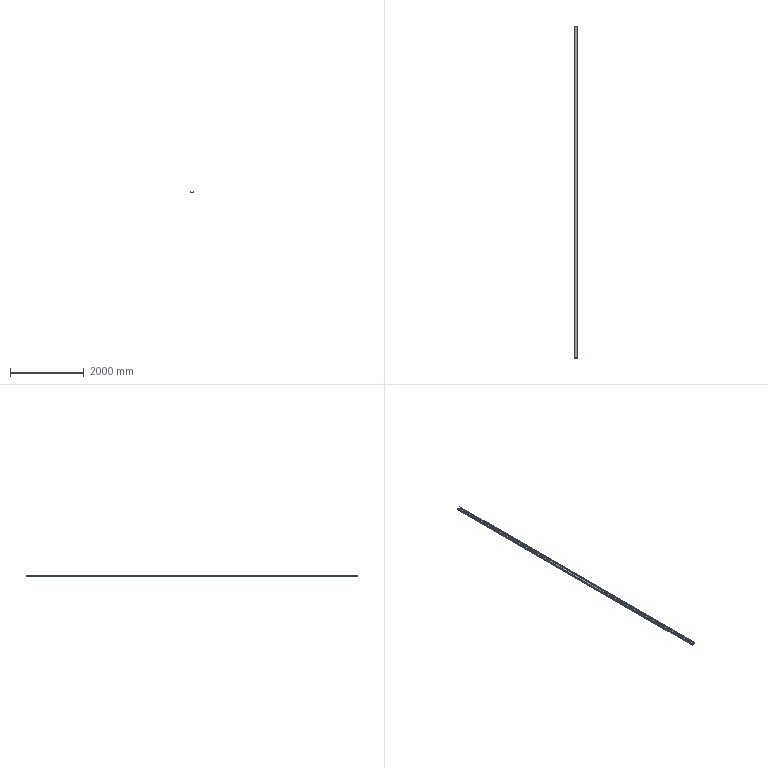Component | NX | CHUNSHUIJINCAO_CAOGANG1 | 1 solid | 10 faces | box 100 x 9000 x 48 mm | volume 11303100 mm3 | plane 10
STEP:
#1=CARTESIAN_POINT('',(0.,0.,0.));
#2=DIRECTION('',(0.,0.,1.));
#3=DIRECTION('',(1.,0.,0.));
#4=AXIS2_PLACEMENT_3D('',#1,#2,#3);
#5=CARTESIAN_POINT('',(2850.,250.,8375.));
#6=VERTEX_POINT('',#5);
#7=CARTESIAN_POINT('',(2850.,250.,8327.));
#8=VERTEX_POINT('',#7);
#9=CARTESIAN_POINT('',(2850.,250.,8327.));
#10=DIRECTION('',(-0.,0.,-1.));
#11=VECTOR('',#10,1.);
#12=LINE('',#9,#11);
#13=CARTESIAN_POINT('',(2850.,150.,8327.));
#14=DIRECTION('',(-1.,0.,0.));
#15=DIRECTION('',(-0.,0.,-1.));
#16=AXIS2_PLACEMENT_3D('',#13,#14,#15);
#17=PLANE('',#16);
#18=CARTESIAN_POINT('',(0.,-100.));
#19=DIRECTION('',(1.,0.));
#20=VECTOR('',#19,1.);
#21=LINE('',#18,#20);
#22=(GEOMETRIC_REPRESENTATION_CONTEXT(2)PARAMETRIC_REPRESENTATION_CONTEXT()REPRESENTATION_CONTEXT('',''));
#23=DEFINITIONAL_REPRESENTATION('',(#21),#22);
#24=PCURVE('',#17,#23);
#25=CARTESIAN_POINT('',(2900.,250.,8351.));
#26=DIRECTION('',(0.,1.,0.));
#27=DIRECTION('',(-1.,0.,0.));
#28=AXIS2_PLACEMENT_3D('',#25,#26,#27);
#29=PLANE('',#28);
#30=CARTESIAN_POINT('',(50.,-24.));
#31=DIRECTION('',(0.,-1.));
#32=VECTOR('',#31,1.);
#33=LINE('',#30,#32);
#34=(GEOMETRIC_REPRESENTATION_CONTEXT(2)PARAMETRIC_REPRESENTATION_CONTEXT()REPRESENTATION_CONTEXT('',''));
#35=DEFINITIONAL_REPRESENTATION('',(#33),#34);
#36=PCURVE('',#29,#35);
#37=SURFACE_CURVE('',#12,(#24,#36),.PCURVE_S1.);
#38=EDGE_CURVE('',#6,#8,#37,.T.);
#39=ORIENTED_EDGE('',*,*,#38,.F.);
#40=CARTESIAN_POINT('',(2850.,9250.,8375.));
#41=VERTEX_POINT('',#40);
#42=CARTESIAN_POINT('',(2850.,150.,8375.));
#43=DIRECTION('',(0.,1.,0.));
#44=VECTOR('',#43,1.);
#45=LINE('',#42,#44);
#46=CARTESIAN_POINT('',(-48.,0.));
#47=DIRECTION('',(0.,-1.));
#48=VECTOR('',#47,1.);
#49=LINE('',#46,#48);
#50=(GEOMETRIC_REPRESENTATION_CONTEXT(2)PARAMETRIC_REPRESENTATION_CONTEXT()REPRESENTATION_CONTEXT('',''));
#51=DEFINITIONAL_REPRESENTATION('',(#49),#50);
#52=PCURVE('',#17,#51);
#53=CARTESIAN_POINT('',(2850.,150.,8375.));
#54=DIRECTION('',(0.,0.,1.));
#55=DIRECTION('',(0.,-1.,0.));
#56=AXIS2_PLACEMENT_3D('',#53,#54,#55);
#57=PLANE('',#56);
#58=CARTESIAN_POINT('',(0.,0.));
#59=DIRECTION('',(-1.,0.));
#60=VECTOR('',#59,1.);
#61=LINE('',#58,#60);
#62=(GEOMETRIC_REPRESENTATION_CONTEXT(2)PARAMETRIC_REPRESENTATION_CONTEXT()REPRESENTATION_CONTEXT('',''));
#63=DEFINITIONAL_REPRESENTATION('',(#61),#62);
#64=PCURVE('',#57,#63);
#65=SURFACE_CURVE('',#45,(#52,#64),.PCURVE_S1.);
#66=EDGE_CURVE('',#6,#41,#65,.T.);
#67=ORIENTED_EDGE('',*,*,#66,.T.);
#68=CARTESIAN_POINT('',(2850.,9250.,8327.));
#69=VERTEX_POINT('',#68);
#70=CARTESIAN_POINT('',(2850.,9250.,8327.));
#71=DIRECTION('',(0.,0.,1.));
#72=VECTOR('',#71,1.);
#73=LINE('',#70,#72);
#74=CARTESIAN_POINT('',(0.,-9100.));
#75=DIRECTION('',(-1.,0.));
#76=VECTOR('',#75,1.);
#77=LINE('',#74,#76);
#78=(GEOMETRIC_REPRESENTATION_CONTEXT(2)PARAMETRIC_REPRESENTATION_CONTEXT()REPRESENTATION_CONTEXT('',''));
#79=DEFINITIONAL_REPRESENTATION('',(#77),#78);
#80=PCURVE('',#17,#79);
#81=CARTESIAN_POINT('',(2900.,9250.,8351.));
#82=DIRECTION('',(0.,-1.,0.));
#83=DIRECTION('',(1.,0.,0.));
#84=AXIS2_PLACEMENT_3D('',#81,#82,#83);
#85=PLANE('',#84);
#86=CARTESIAN_POINT('',(-50.,-24.));
#87=DIRECTION('',(0.,1.));
#88=VECTOR('',#87,1.);
#89=LINE('',#86,#88);
#90=(GEOMETRIC_REPRESENTATION_CONTEXT(2)PARAMETRIC_REPRESENTATION_CONTEXT()REPRESENTATION_CONTEXT('',''));
#91=DEFINITIONAL_REPRESENTATION('',(#89),#90);
#92=PCURVE('',#85,#91);
#93=SURFACE_CURVE('',#73,(#80,#92),.PCURVE_S1.);
#94=EDGE_CURVE('',#69,#41,#93,.T.);
#95=ORIENTED_EDGE('',*,*,#94,.F.);
#96=CARTESIAN_POINT('',(2850.,150.,8327.));
#97=DIRECTION('',(0.,1.,0.));
#98=VECTOR('',#97,1.);
#99=LINE('',#96,#98);
#100=CARTESIAN_POINT('',(0.,0.));
#101=DIRECTION('',(0.,-1.));
#102=VECTOR('',#101,1.);
#103=LINE('',#100,#102);
#104=(GEOMETRIC_REPRESENTATION_CONTEXT(2)PARAMETRIC_REPRESENTATION_CONTEXT()REPRESENTATION_CONTEXT('',''));
#105=DEFINITIONAL_REPRESENTATION('',(#103),#104);
#106=PCURVE('',#17,#105);
#107=CARTESIAN_POINT('',(2950.,150.,8327.));
#108=DIRECTION('',(0.,0.,-1.));
#109=DIRECTION('',(0.,1.,0.));
#110=AXIS2_PLACEMENT_3D('',#107,#108,#109);
#111=PLANE('',#110);
#112=CARTESIAN_POINT('',(0.,-100.));
#113=DIRECTION('',(1.,0.));
#114=VECTOR('',#113,1.);
#115=LINE('',#112,#114);
#116=(GEOMETRIC_REPRESENTATION_CONTEXT(2)PARAMETRIC_REPRESENTATION_CONTEXT()REPRESENTATION_CONTEXT('',''));
#117=DEFINITIONAL_REPRESENTATION('',(#115),#116);
#118=PCURVE('',#111,#117);
#119=SURFACE_CURVE('',#99,(#106,#118),.PCURVE_S1.);
#120=EDGE_CURVE('',#8,#69,#119,.T.);
#121=ORIENTED_EDGE('',*,*,#120,.F.);
#122=EDGE_LOOP('',(#39,#67,#95,#121));
#123=FACE_BOUND('',#122,.T.);
#124=ADVANCED_FACE('',(#123),#17,.T.);
#125=CARTESIAN_POINT('',(2858.5,250.,8375.));
#126=VERTEX_POINT('',#125);
#127=CARTESIAN_POINT('',(2850.,250.,8375.));
#128=DIRECTION('',(-1.,0.,0.));
#129=VECTOR('',#128,1.);
#130=LINE('',#127,#129);
#131=CARTESIAN_POINT('',(-100.,0.));
#132=DIRECTION('',(0.,-1.));
#133=VECTOR('',#132,1.);
#134=LINE('',#131,#133);
#135=(GEOMETRIC_REPRESENTATION_CONTEXT(2)PARAMETRIC_REPRESENTATION_CONTEXT()REPRESENTATION_CONTEXT('',''));
#136=DEFINITIONAL_REPRESENTATION('',(#134),#135);
#137=PCURVE('',#57,#136);
#138=CARTESIAN_POINT('',(50.,24.));
#139=DIRECTION('',(1.,0.));
#140=VECTOR('',#139,1.);
#141=LINE('',#138,#140);
#142=(GEOMETRIC_REPRESENTATION_CONTEXT(2)PARAMETRIC_REPRESENTATION_CONTEXT()REPRESENTATION_CONTEXT('',''));
#143=DEFINITIONAL_REPRESENTATION('',(#141),#142);
#144=PCURVE('',#29,#143);
#145=SURFACE_CURVE('',#130,(#137,#144),.PCURVE_S1.);
#146=EDGE_CURVE('',#126,#6,#145,.T.);
#147=ORIENTED_EDGE('',*,*,#146,.F.);
#148=CARTESIAN_POINT('',(2858.5,9250.,8375.));
#149=VERTEX_POINT('',#148);
#150=CARTESIAN_POINT('',(2858.5,150.,8375.));
#151=DIRECTION('',(0.,1.,0.));
#152=VECTOR('',#151,1.);
#153=LINE('',#150,#152);
#154=CARTESIAN_POINT('',(0.,8.5));
#155=DIRECTION('',(-1.,0.));
#156=VECTOR('',#155,1.);
#157=LINE('',#154,#156);
#158=(GEOMETRIC_REPRESENTATION_CONTEXT(2)PARAMETRIC_REPRESENTATION_CONTEXT()REPRESENTATION_CONTEXT('',''));
#159=DEFINITIONAL_REPRESENTATION('',(#157),#158);
#160=PCURVE('',#57,#159);
#161=CARTESIAN_POINT('',(2858.5,150.,8375.));
#162=DIRECTION('',(1.,0.,-0.));
#163=DIRECTION('',(0.,0.,1.));
#164=AXIS2_PLACEMENT_3D('',#161,#162,#163);
#165=PLANE('',#164);
#166=CARTESIAN_POINT('',(0.,0.));
#167=DIRECTION('',(0.,-1.));
#168=VECTOR('',#167,1.);
#169=LINE('',#166,#168);
#170=(GEOMETRIC_REPRESENTATION_CONTEXT(2)PARAMETRIC_REPRESENTATION_CONTEXT()REPRESENTATION_CONTEXT('',''));
#171=DEFINITIONAL_REPRESENTATION('',(#169),#170);
#172=PCURVE('',#165,#171);
#173=SURFACE_CURVE('',#153,(#160,#172),.PCURVE_S1.);
#174=EDGE_CURVE('',#126,#149,#173,.T.);
#175=ORIENTED_EDGE('',*,*,#174,.T.);
#176=CARTESIAN_POINT('',(2850.,9250.,8375.));
#177=DIRECTION('',(1.,0.,0.));
#178=VECTOR('',#177,1.);
#179=LINE('',#176,#178);
#180=CARTESIAN_POINT('',(-9100.,0.));
#181=DIRECTION('',(0.,1.));
#182=VECTOR('',#181,1.);
#183=LINE('',#180,#182);
#184=(GEOMETRIC_REPRESENTATION_CONTEXT(2)PARAMETRIC_REPRESENTATION_CONTEXT()REPRESENTATION_CONTEXT('',''));
#185=DEFINITIONAL_REPRESENTATION('',(#183),#184);
#186=PCURVE('',#57,#185);
#187=CARTESIAN_POINT('',(-50.,24.));
#188=DIRECTION('',(1.,0.));
#189=VECTOR('',#188,1.);
#190=LINE('',#187,#189);
#191=(GEOMETRIC_REPRESENTATION_CONTEXT(2)PARAMETRIC_REPRESENTATION_CONTEXT()REPRESENTATION_CONTEXT('',''));
#192=DEFINITIONAL_REPRESENTATION('',(#190),#191);
#193=PCURVE('',#85,#192);
#194=SURFACE_CURVE('',#179,(#186,#193),.PCURVE_S1.);
#195=EDGE_CURVE('',#41,#149,#194,.T.);
#196=ORIENTED_EDGE('',*,*,#195,.F.);
#197=ORIENTED_EDGE('',*,*,#66,.F.);
#198=EDGE_LOOP('',(#147,#175,#196,#197));
#199=FACE_BOUND('',#198,.T.);
#200=ADVANCED_FACE('',(#199),#57,.T.);
#201=CARTESIAN_POINT('',(2858.5,250.,8332.3));
#202=VERTEX_POINT('',#201);
#203=CARTESIAN_POINT('',(2858.5,250.,8375.));
#204=DIRECTION('',(0.,0.,1.));
#205=VECTOR('',#204,1.);
#206=LINE('',#203,#205);
#207=CARTESIAN_POINT('',(0.,-100.));
#208=DIRECTION('',(1.,0.));
#209=VECTOR('',#208,1.);
#210=LINE('',#207,#209);
#211=(GEOMETRIC_REPRESENTATION_CONTEXT(2)PARAMETRIC_REPRESENTATION_CONTEXT()REPRESENTATION_CONTEXT('',''));
#212=DEFINITIONAL_REPRESENTATION('',(#210),#211);
#213=PCURVE('',#165,#212);
#214=CARTESIAN_POINT('',(41.5,24.));
#215=DIRECTION('',(-0.,1.));
#216=VECTOR('',#215,1.);
#217=LINE('',#214,#216);
#218=(GEOMETRIC_REPRESENTATION_CONTEXT(2)PARAMETRIC_REPRESENTATION_CONTEXT()REPRESENTATION_CONTEXT('',''));
#219=DEFINITIONAL_REPRESENTATION('',(#217),#218);
#220=PCURVE('',#29,#219);
#221=SURFACE_CURVE('',#206,(#213,#220),.PCURVE_S1.);
#222=EDGE_CURVE('',#202,#126,#221,.T.);
#223=ORIENTED_EDGE('',*,*,#222,.F.);
#224=CARTESIAN_POINT('',(2858.5,9250.,8332.3));
#225=VERTEX_POINT('',#224);
#226=CARTESIAN_POINT('',(2858.5,150.,8332.3));
#227=DIRECTION('',(0.,1.,0.));
#228=VECTOR('',#227,1.);
#229=LINE('',#226,#228);
#230=CARTESIAN_POINT('',(-42.7,0.));
#231=DIRECTION('',(0.,-1.));
#232=VECTOR('',#231,1.);
#233=LINE('',#230,#232);
#234=(GEOMETRIC_REPRESENTATION_CONTEXT(2)PARAMETRIC_REPRESENTATION_CONTEXT()REPRESENTATION_CONTEXT('',''));
#235=DEFINITIONAL_REPRESENTATION('',(#233),#234);
#236=PCURVE('',#165,#235);
#237=CARTESIAN_POINT('',(2900.,150.,8332.3));
#238=DIRECTION('',(0.,0.,1.));
#239=DIRECTION('',(0.,-1.,0.));
#240=AXIS2_PLACEMENT_3D('',#237,#238,#239);
#241=PLANE('',#240);
#242=CARTESIAN_POINT('',(0.,-41.5));
#243=DIRECTION('',(-1.,0.));
#244=VECTOR('',#243,1.);
#245=LINE('',#242,#244);
#246=(GEOMETRIC_REPRESENTATION_CONTEXT(2)PARAMETRIC_REPRESENTATION_CONTEXT()REPRESENTATION_CONTEXT('',''));
#247=DEFINITIONAL_REPRESENTATION('',(#245),#246);
#248=PCURVE('',#241,#247);
#249=SURFACE_CURVE('',#229,(#236,#248),.PCURVE_S1.);
#250=EDGE_CURVE('',#202,#225,#249,.T.);
#251=ORIENTED_EDGE('',*,*,#250,.T.);
#252=CARTESIAN_POINT('',(2858.5,9250.,8375.));
#253=DIRECTION('',(-0.,0.,-1.));
#254=VECTOR('',#253,1.);
#255=LINE('',#252,#254);
#256=CARTESIAN_POINT('',(0.,-9100.));
#257=DIRECTION('',(-1.,0.));
#258=VECTOR('',#257,1.);
#259=LINE('',#256,#258);
#260=(GEOMETRIC_REPRESENTATION_CONTEXT(2)PARAMETRIC_REPRESENTATION_CONTEXT()REPRESENTATION_CONTEXT('',''));
#261=DEFINITIONAL_REPRESENTATION('',(#259),#260);
#262=PCURVE('',#165,#261);
#263=CARTESIAN_POINT('',(-41.5,24.));
#264=DIRECTION('',(-0.,-1.));
#265=VECTOR('',#264,1.);
#266=LINE('',#263,#265);
#267=(GEOMETRIC_REPRESENTATION_CONTEXT(2)PARAMETRIC_REPRESENTATION_CONTEXT()REPRESENTATION_CONTEXT('',''));
#268=DEFINITIONAL_REPRESENTATION('',(#266),#267);
#269=PCURVE('',#85,#268);
#270=SURFACE_CURVE('',#255,(#262,#269),.PCURVE_S1.);
#271=EDGE_CURVE('',#149,#225,#270,.T.);
#272=ORIENTED_EDGE('',*,*,#271,.F.);
#273=ORIENTED_EDGE('',*,*,#174,.F.);
#274=EDGE_LOOP('',(#223,#251,#272,#273));
#275=FACE_BOUND('',#274,.T.);
#276=ADVANCED_FACE('',(#275),#165,.T.);
#277=CARTESIAN_POINT('',(2941.5,250.,8332.3));
#278=VERTEX_POINT('',#277);
#279=CARTESIAN_POINT('',(2900.,250.,8332.3));
#280=DIRECTION('',(-1.,0.,0.));
#281=VECTOR('',#280,1.);
#282=LINE('',#279,#281);
#283=CARTESIAN_POINT('',(-100.,0.));
#284=DIRECTION('',(0.,-1.));
#285=VECTOR('',#284,1.);
#286=LINE('',#283,#285);
#287=(GEOMETRIC_REPRESENTATION_CONTEXT(2)PARAMETRIC_REPRESENTATION_CONTEXT()REPRESENTATION_CONTEXT('',''));
#288=DEFINITIONAL_REPRESENTATION('',(#286),#287);
#289=PCURVE('',#241,#288);
#290=CARTESIAN_POINT('',(0.,-18.7));
#291=DIRECTION('',(1.,0.));
#292=VECTOR('',#291,1.);
#293=LINE('',#290,#292);
#294=(GEOMETRIC_REPRESENTATION_CONTEXT(2)PARAMETRIC_REPRESENTATION_CONTEXT()REPRESENTATION_CONTEXT('',''));
#295=DEFINITIONAL_REPRESENTATION('',(#293),#294);
#296=PCURVE('',#29,#295);
#297=SURFACE_CURVE('',#282,(#289,#296),.PCURVE_S1.);
#298=EDGE_CURVE('',#278,#202,#297,.T.);
#299=ORIENTED_EDGE('',*,*,#298,.F.);
#300=CARTESIAN_POINT('',(2941.5,9250.,8332.3));
#301=VERTEX_POINT('',#300);
#302=CARTESIAN_POINT('',(2941.5,150.,8332.3));
#303=DIRECTION('',(0.,1.,0.));
#304=VECTOR('',#303,1.);
#305=LINE('',#302,#304);
#306=CARTESIAN_POINT('',(0.,41.5));
#307=DIRECTION('',(-1.,0.));
#308=VECTOR('',#307,1.);
#309=LINE('',#306,#308);
#310=(GEOMETRIC_REPRESENTATION_CONTEXT(2)PARAMETRIC_REPRESENTATION_CONTEXT()REPRESENTATION_CONTEXT('',''));
#311=DEFINITIONAL_REPRESENTATION('',(#309),#310);
#312=PCURVE('',#241,#311);
#313=CARTESIAN_POINT('',(2941.5,150.,8332.3));
#314=DIRECTION('',(-1.,0.,0.));
#315=DIRECTION('',(-0.,0.,-1.));
#316=AXIS2_PLACEMENT_3D('',#313,#314,#315);
#317=PLANE('',#316);
#318=CARTESIAN_POINT('',(0.,0.));
#319=DIRECTION('',(0.,-1.));
#320=VECTOR('',#319,1.);
#321=LINE('',#318,#320);
#322=(GEOMETRIC_REPRESENTATION_CONTEXT(2)PARAMETRIC_REPRESENTATION_CONTEXT()REPRESENTATION_CONTEXT('',''));
#323=DEFINITIONAL_REPRESENTATION('',(#321),#322);
#324=PCURVE('',#317,#323);
#325=SURFACE_CURVE('',#305,(#312,#324),.PCURVE_S1.);
#326=EDGE_CURVE('',#278,#301,#325,.T.);
#327=ORIENTED_EDGE('',*,*,#326,.T.);
#328=CARTESIAN_POINT('',(2900.,9250.,8332.3));
#329=DIRECTION('',(1.,0.,0.));
#330=VECTOR('',#329,1.);
#331=LINE('',#328,#330);
#332=CARTESIAN_POINT('',(-9100.,0.));
#333=DIRECTION('',(0.,1.));
#334=VECTOR('',#333,1.);
#335=LINE('',#332,#334);
#336=(GEOMETRIC_REPRESENTATION_CONTEXT(2)PARAMETRIC_REPRESENTATION_CONTEXT()REPRESENTATION_CONTEXT('',''));
#337=DEFINITIONAL_REPRESENTATION('',(#335),#336);
#338=PCURVE('',#241,#337);
#339=CARTESIAN_POINT('',(0.,-18.7));
#340=DIRECTION('',(1.,0.));
#341=VECTOR('',#340,1.);
#342=LINE('',#339,#341);
#343=(GEOMETRIC_REPRESENTATION_CONTEXT(2)PARAMETRIC_REPRESENTATION_CONTEXT()REPRESENTATION_CONTEXT('',''));
#344=DEFINITIONAL_REPRESENTATION('',(#342),#343);
#345=PCURVE('',#85,#344);
#346=SURFACE_CURVE('',#331,(#338,#345),.PCURVE_S1.);
#347=EDGE_CURVE('',#225,#301,#346,.T.);
#348=ORIENTED_EDGE('',*,*,#347,.F.);
#349=ORIENTED_EDGE('',*,*,#250,.F.);
#350=EDGE_LOOP('',(#299,#327,#348,#349));
#351=FACE_BOUND('',#350,.T.);
#352=ADVANCED_FACE('',(#351),#241,.T.);
#353=CARTESIAN_POINT('',(2941.5,250.,8375.));
#354=VERTEX_POINT('',#353);
#355=CARTESIAN_POINT('',(2941.5,250.,8332.3));
#356=DIRECTION('',(-0.,0.,-1.));
#357=VECTOR('',#356,1.);
#358=LINE('',#355,#357);
#359=CARTESIAN_POINT('',(0.,-100.));
#360=DIRECTION('',(1.,0.));
#361=VECTOR('',#360,1.);
#362=LINE('',#359,#361);
#363=(GEOMETRIC_REPRESENTATION_CONTEXT(2)PARAMETRIC_REPRESENTATION_CONTEXT()REPRESENTATION_CONTEXT('',''));
#364=DEFINITIONAL_REPRESENTATION('',(#362),#363);
#365=PCURVE('',#317,#364);
#366=CARTESIAN_POINT('',(-41.5,-18.7));
#367=DIRECTION('',(0.,-1.));
#368=VECTOR('',#367,1.);
#369=LINE('',#366,#368);
#370=(GEOMETRIC_REPRESENTATION_CONTEXT(2)PARAMETRIC_REPRESENTATION_CONTEXT()REPRESENTATION_CONTEXT('',''));
#371=DEFINITIONAL_REPRESENTATION('',(#369),#370);
#372=PCURVE('',#29,#371);
#373=SURFACE_CURVE('',#358,(#365,#372),.PCURVE_S1.);
#374=EDGE_CURVE('',#354,#278,#373,.T.);
#375=ORIENTED_EDGE('',*,*,#374,.F.);
#376=CARTESIAN_POINT('',(2941.5,9250.,8375.));
#377=VERTEX_POINT('',#376);
#378=CARTESIAN_POINT('',(2941.5,150.,8375.));
#379=DIRECTION('',(0.,1.,0.));
#380=VECTOR('',#379,1.);
#381=LINE('',#378,#380);
#382=CARTESIAN_POINT('',(-42.7,0.));
#383=DIRECTION('',(0.,-1.));
#384=VECTOR('',#383,1.);
#385=LINE('',#382,#384);
#386=(GEOMETRIC_REPRESENTATION_CONTEXT(2)PARAMETRIC_REPRESENTATION_CONTEXT()REPRESENTATION_CONTEXT('',''));
#387=DEFINITIONAL_REPRESENTATION('',(#385),#386);
#388=PCURVE('',#317,#387);
#389=CARTESIAN_POINT('',(2941.5,150.,8375.));
#390=DIRECTION('',(0.,0.,1.));
#391=DIRECTION('',(-1.,0.,0.));
#392=AXIS2_PLACEMENT_3D('',#389,#390,#391);
#393=PLANE('',#392);
#394=CARTESIAN_POINT('',(0.,0.));
#395=DIRECTION('',(0.,-1.));
#396=VECTOR('',#395,1.);
#397=LINE('',#394,#396);
#398=(GEOMETRIC_REPRESENTATION_CONTEXT(2)PARAMETRIC_REPRESENTATION_CONTEXT()REPRESENTATION_CONTEXT('',''));
#399=DEFINITIONAL_REPRESENTATION('',(#397),#398);
#400=PCURVE('',#393,#399);
#401=SURFACE_CURVE('',#381,(#388,#400),.PCURVE_S1.);
#402=EDGE_CURVE('',#354,#377,#401,.T.);
#403=ORIENTED_EDGE('',*,*,#402,.T.);
#404=CARTESIAN_POINT('',(2941.5,9250.,8332.3));
#405=DIRECTION('',(0.,0.,1.));
#406=VECTOR('',#405,1.);
#407=LINE('',#404,#406);
#408=CARTESIAN_POINT('',(0.,-9100.));
#409=DIRECTION('',(-1.,0.));
#410=VECTOR('',#409,1.);
#411=LINE('',#408,#410);
#412=(GEOMETRIC_REPRESENTATION_CONTEXT(2)PARAMETRIC_REPRESENTATION_CONTEXT()REPRESENTATION_CONTEXT('',''));
#413=DEFINITIONAL_REPRESENTATION('',(#411),#412);
#414=PCURVE('',#317,#413);
#415=CARTESIAN_POINT('',(41.5,-18.7));
#416=DIRECTION('',(0.,1.));
#417=VECTOR('',#416,1.);
#418=LINE('',#415,#417);
#419=(GEOMETRIC_REPRESENTATION_CONTEXT(2)PARAMETRIC_REPRESENTATION_CONTEXT()REPRESENTATION_CONTEXT('',''));
#420=DEFINITIONAL_REPRESENTATION('',(#418),#419);
#421=PCURVE('',#85,#420);
#422=SURFACE_CURVE('',#407,(#414,#421),.PCURVE_S1.);
#423=EDGE_CURVE('',#301,#377,#422,.T.);
#424=ORIENTED_EDGE('',*,*,#423,.F.);
#425=ORIENTED_EDGE('',*,*,#326,.F.);
#426=EDGE_LOOP('',(#375,#403,#424,#425));
#427=FACE_BOUND('',#426,.T.);
#428=ADVANCED_FACE('',(#427),#317,.T.);
#429=CARTESIAN_POINT('',(2950.,250.,8375.));
#430=VERTEX_POINT('',#429);
#431=CARTESIAN_POINT('',(2941.5,250.,8375.));
#432=DIRECTION('',(-1.,0.,0.));
#433=VECTOR('',#432,1.);
#434=LINE('',#431,#433);
#435=CARTESIAN_POINT('',(0.,-100.));
#436=DIRECTION('',(1.,0.));
#437=VECTOR('',#436,1.);
#438=LINE('',#435,#437);
#439=(GEOMETRIC_REPRESENTATION_CONTEXT(2)PARAMETRIC_REPRESENTATION_CONTEXT()REPRESENTATION_CONTEXT('',''));
#440=DEFINITIONAL_REPRESENTATION('',(#438),#439);
#441=PCURVE('',#393,#440);
#442=CARTESIAN_POINT('',(-41.5,24.));
#443=DIRECTION('',(1.,0.));
#444=VECTOR('',#443,1.);
#445=LINE('',#442,#444);
#446=(GEOMETRIC_REPRESENTATION_CONTEXT(2)PARAMETRIC_REPRESENTATION_CONTEXT()REPRESENTATION_CONTEXT('',''));
#447=DEFINITIONAL_REPRESENTATION('',(#445),#446);
#448=PCURVE('',#29,#447);
#449=SURFACE_CURVE('',#434,(#441,#448),.PCURVE_S1.);
#450=EDGE_CURVE('',#430,#354,#449,.T.);
#451=ORIENTED_EDGE('',*,*,#450,.F.);
#452=CARTESIAN_POINT('',(2950.,9250.,8375.));
#453=VERTEX_POINT('',#452);
#454=CARTESIAN_POINT('',(2950.,150.,8375.));
#455=DIRECTION('',(0.,1.,0.));
#456=VECTOR('',#455,1.);
#457=LINE('',#454,#456);
#458=CARTESIAN_POINT('',(-8.5,0.));
#459=DIRECTION('',(0.,-1.));
#460=VECTOR('',#459,1.);
#461=LINE('',#458,#460);
#462=(GEOMETRIC_REPRESENTATION_CONTEXT(2)PARAMETRIC_REPRESENTATION_CONTEXT()REPRESENTATION_CONTEXT('',''));
#463=DEFINITIONAL_REPRESENTATION('',(#461),#462);
#464=PCURVE('',#393,#463);
#465=CARTESIAN_POINT('',(2950.,150.,8375.));
#466=DIRECTION('',(1.,0.,-0.));
#467=DIRECTION('',(0.,0.,1.));
#468=AXIS2_PLACEMENT_3D('',#465,#466,#467);
#469=PLANE('',#468);
#470=CARTESIAN_POINT('',(0.,0.));
#471=DIRECTION('',(0.,-1.));
#472=VECTOR('',#471,1.);
#473=LINE('',#470,#472);
#474=(GEOMETRIC_REPRESENTATION_CONTEXT(2)PARAMETRIC_REPRESENTATION_CONTEXT()REPRESENTATION_CONTEXT('',''));
#475=DEFINITIONAL_REPRESENTATION('',(#473),#474);
#476=PCURVE('',#469,#475);
#477=SURFACE_CURVE('',#457,(#464,#476),.PCURVE_S1.);
#478=EDGE_CURVE('',#430,#453,#477,.T.);
#479=ORIENTED_EDGE('',*,*,#478,.T.);
#480=CARTESIAN_POINT('',(2941.5,9250.,8375.));
#481=DIRECTION('',(1.,0.,-0.));
#482=VECTOR('',#481,1.);
#483=LINE('',#480,#482);
#484=CARTESIAN_POINT('',(0.,-9100.));
#485=DIRECTION('',(-1.,0.));
#486=VECTOR('',#485,1.);
#487=LINE('',#484,#486);
#488=(GEOMETRIC_REPRESENTATION_CONTEXT(2)PARAMETRIC_REPRESENTATION_CONTEXT()REPRESENTATION_CONTEXT('',''));
#489=DEFINITIONAL_REPRESENTATION('',(#487),#488);
#490=PCURVE('',#393,#489);
#491=CARTESIAN_POINT('',(41.5,24.));
#492=DIRECTION('',(1.,-0.));
#493=VECTOR('',#492,1.);
#494=LINE('',#491,#493);
#495=(GEOMETRIC_REPRESENTATION_CONTEXT(2)PARAMETRIC_REPRESENTATION_CONTEXT()REPRESENTATION_CONTEXT('',''));
#496=DEFINITIONAL_REPRESENTATION('',(#494),#495);
#497=PCURVE('',#85,#496);
#498=SURFACE_CURVE('',#483,(#490,#497),.PCURVE_S1.);
#499=EDGE_CURVE('',#377,#453,#498,.T.);
#500=ORIENTED_EDGE('',*,*,#499,.F.);
#501=ORIENTED_EDGE('',*,*,#402,.F.);
#502=EDGE_LOOP('',(#451,#479,#500,#501));
#503=FACE_BOUND('',#502,.T.);
#504=ADVANCED_FACE('',(#503),#393,.T.);
#505=CARTESIAN_POINT('',(2950.,250.,8327.));
#506=VERTEX_POINT('',#505);
#507=CARTESIAN_POINT('',(2950.,250.,8375.));
#508=DIRECTION('',(0.,0.,1.));
#509=VECTOR('',#508,1.);
#510=LINE('',#507,#509);
#511=CARTESIAN_POINT('',(0.,-100.));
#512=DIRECTION('',(1.,0.));
#513=VECTOR('',#512,1.);
#514=LINE('',#511,#513);
#515=(GEOMETRIC_REPRESENTATION_CONTEXT(2)PARAMETRIC_REPRESENTATION_CONTEXT()REPRESENTATION_CONTEXT('',''));
#516=DEFINITIONAL_REPRESENTATION('',(#514),#515);
#517=PCURVE('',#469,#516);
#518=CARTESIAN_POINT('',(-50.,24.));
#519=DIRECTION('',(-0.,1.));
#520=VECTOR('',#519,1.);
#521=LINE('',#518,#520);
#522=(GEOMETRIC_REPRESENTATION_CONTEXT(2)PARAMETRIC_REPRESENTATION_CONTEXT()REPRESENTATION_CONTEXT('',''));
#523=DEFINITIONAL_REPRESENTATION('',(#521),#522);
#524=PCURVE('',#29,#523);
#525=SURFACE_CURVE('',#510,(#517,#524),.PCURVE_S1.);
#526=EDGE_CURVE('',#506,#430,#525,.T.);
#527=ORIENTED_EDGE('',*,*,#526,.F.);
#528=CARTESIAN_POINT('',(2950.,9250.,8327.));
#529=VERTEX_POINT('',#528);
#530=CARTESIAN_POINT('',(2950.,150.,8327.));
#531=DIRECTION('',(0.,1.,0.));
#532=VECTOR('',#531,1.);
#533=LINE('',#530,#532);
#534=CARTESIAN_POINT('',(-48.,0.));
#535=DIRECTION('',(0.,-1.));
#536=VECTOR('',#535,1.);
#537=LINE('',#534,#536);
#538=(GEOMETRIC_REPRESENTATION_CONTEXT(2)PARAMETRIC_REPRESENTATION_CONTEXT()REPRESENTATION_CONTEXT('',''));
#539=DEFINITIONAL_REPRESENTATION('',(#537),#538);
#540=PCURVE('',#469,#539);
#541=CARTESIAN_POINT('',(0.,0.));
#542=DIRECTION('',(1.,0.));
#543=VECTOR('',#542,1.);
#544=LINE('',#541,#543);
#545=(GEOMETRIC_REPRESENTATION_CONTEXT(2)PARAMETRIC_REPRESENTATION_CONTEXT()REPRESENTATION_CONTEXT('',''));
#546=DEFINITIONAL_REPRESENTATION('',(#544),#545);
#547=PCURVE('',#111,#546);
#548=SURFACE_CURVE('',#533,(#540,#547),.PCURVE_S1.);
#549=EDGE_CURVE('',#506,#529,#548,.T.);
#550=ORIENTED_EDGE('',*,*,#549,.T.);
#551=CARTESIAN_POINT('',(2950.,9250.,8375.));
#552=DIRECTION('',(-0.,0.,-1.));
#553=VECTOR('',#552,1.);
#554=LINE('',#551,#553);
#555=CARTESIAN_POINT('',(0.,-9100.));
#556=DIRECTION('',(-1.,0.));
#557=VECTOR('',#556,1.);
#558=LINE('',#555,#557);
#559=(GEOMETRIC_REPRESENTATION_CONTEXT(2)PARAMETRIC_REPRESENTATION_CONTEXT()REPRESENTATION_CONTEXT('',''));
#560=DEFINITIONAL_REPRESENTATION('',(#558),#559);
#561=PCURVE('',#469,#560);
#562=CARTESIAN_POINT('',(50.,24.));
#563=DIRECTION('',(-0.,-1.));
#564=VECTOR('',#563,1.);
#565=LINE('',#562,#564);
#566=(GEOMETRIC_REPRESENTATION_CONTEXT(2)PARAMETRIC_REPRESENTATION_CONTEXT()REPRESENTATION_CONTEXT('',''));
#567=DEFINITIONAL_REPRESENTATION('',(#565),#566);
#568=PCURVE('',#85,#567);
#569=SURFACE_CURVE('',#554,(#561,#568),.PCURVE_S1.);
#570=EDGE_CURVE('',#453,#529,#569,.T.);
#571=ORIENTED_EDGE('',*,*,#570,.F.);
#572=ORIENTED_EDGE('',*,*,#478,.F.);
#573=EDGE_LOOP('',(#527,#550,#571,#572));
#574=FACE_BOUND('',#573,.T.);
#575=ADVANCED_FACE('',(#574),#469,.T.);
#576=CARTESIAN_POINT('',(2950.,250.,8327.));
#577=DIRECTION('',(1.,0.,0.));
#578=VECTOR('',#577,1.);
#579=LINE('',#576,#578);
#580=CARTESIAN_POINT('',(100.,0.));
#581=DIRECTION('',(0.,1.));
#582=VECTOR('',#581,1.);
#583=LINE('',#580,#582);
#584=(GEOMETRIC_REPRESENTATION_CONTEXT(2)PARAMETRIC_REPRESENTATION_CONTEXT()REPRESENTATION_CONTEXT('',''));
#585=DEFINITIONAL_REPRESENTATION('',(#583),#584);
#586=PCURVE('',#111,#585);
#587=CARTESIAN_POINT('',(-50.,-24.));
#588=DIRECTION('',(-1.,0.));
#589=VECTOR('',#588,1.);
#590=LINE('',#587,#589);
#591=(GEOMETRIC_REPRESENTATION_CONTEXT(2)PARAMETRIC_REPRESENTATION_CONTEXT()REPRESENTATION_CONTEXT('',''));
#592=DEFINITIONAL_REPRESENTATION('',(#590),#591);
#593=PCURVE('',#29,#592);
#594=SURFACE_CURVE('',#579,(#586,#593),.PCURVE_S1.);
#595=EDGE_CURVE('',#8,#506,#594,.T.);
#596=ORIENTED_EDGE('',*,*,#595,.F.);
#597=ORIENTED_EDGE('',*,*,#120,.T.);
#598=CARTESIAN_POINT('',(2950.,9250.,8327.));
#599=DIRECTION('',(-1.,0.,0.));
#600=VECTOR('',#599,1.);
#601=LINE('',#598,#600);
#602=CARTESIAN_POINT('',(9100.,0.));
#603=DIRECTION('',(0.,-1.));
#604=VECTOR('',#603,1.);
#605=LINE('',#602,#604);
#606=(GEOMETRIC_REPRESENTATION_CONTEXT(2)PARAMETRIC_REPRESENTATION_CONTEXT()REPRESENTATION_CONTEXT('',''));
#607=DEFINITIONAL_REPRESENTATION('',(#605),#606);
#608=PCURVE('',#111,#607);
#609=CARTESIAN_POINT('',(50.,-24.));
#610=DIRECTION('',(-1.,0.));
#611=VECTOR('',#610,1.);
#612=LINE('',#609,#611);
#613=(GEOMETRIC_REPRESENTATION_CONTEXT(2)PARAMETRIC_REPRESENTATION_CONTEXT()REPRESENTATION_CONTEXT('',''));
#614=DEFINITIONAL_REPRESENTATION('',(#612),#613);
#615=PCURVE('',#85,#614);
#616=SURFACE_CURVE('',#601,(#608,#615),.PCURVE_S1.);
#617=EDGE_CURVE('',#529,#69,#616,.T.);
#618=ORIENTED_EDGE('',*,*,#617,.F.);
#619=ORIENTED_EDGE('',*,*,#549,.F.);
#620=EDGE_LOOP('',(#596,#597,#618,#619));
#621=FACE_BOUND('',#620,.T.);
#622=ADVANCED_FACE('',(#621),#111,.T.);
#623=ORIENTED_EDGE('',*,*,#94,.T.);
#624=ORIENTED_EDGE('',*,*,#195,.T.);
#625=ORIENTED_EDGE('',*,*,#271,.T.);
#626=ORIENTED_EDGE('',*,*,#347,.T.);
#627=ORIENTED_EDGE('',*,*,#423,.T.);
#628=ORIENTED_EDGE('',*,*,#499,.T.);
#629=ORIENTED_EDGE('',*,*,#570,.T.);
#630=ORIENTED_EDGE('',*,*,#617,.T.);
#631=EDGE_LOOP('',(#623,#624,#625,#626,#627,#628,#629,#630));
#632=FACE_BOUND('',#631,.T.);
#633=ADVANCED_FACE('',(#632),#85,.F.);
#634=ORIENTED_EDGE('',*,*,#38,.T.);
#635=ORIENTED_EDGE('',*,*,#595,.T.);
#636=ORIENTED_EDGE('',*,*,#526,.T.);
#637=ORIENTED_EDGE('',*,*,#450,.T.);
#638=ORIENTED_EDGE('',*,*,#374,.T.);
#639=ORIENTED_EDGE('',*,*,#298,.T.);
#640=ORIENTED_EDGE('',*,*,#222,.T.);
#641=ORIENTED_EDGE('',*,*,#146,.T.);
#642=EDGE_LOOP('',(#634,#635,#636,#637,#638,#639,#640,#641));
#643=FACE_BOUND('',#642,.T.);
#644=ADVANCED_FACE('',(#643),#29,.F.);
#645=CLOSED_SHELL('',(#124,#200,#276,#352,#428,#504,#575,#622,#633,#644));
#646=MANIFOLD_SOLID_BREP('',#645);
#647=(LENGTH_UNIT()NAMED_UNIT(*)SI_UNIT(.MILLI.,.METRE.));
#648=UNCERTAINTY_MEASURE_WITH_UNIT(LENGTH_MEASURE(0.0000001),#647,'','');
#649=(NAMED_UNIT(*)PLANE_ANGLE_UNIT()SI_UNIT($,.RADIAN.));
#650=(NAMED_UNIT(*)SI_UNIT($,.STERADIAN.)SOLID_ANGLE_UNIT());
#651=(GEOMETRIC_REPRESENTATION_CONTEXT(3)GLOBAL_UNCERTAINTY_ASSIGNED_CONTEXT((#648))GLOBAL_UNIT_ASSIGNED_CONTEXT((#647,#649,#650))REPRESENTATION_CONTEXT('',''));
#652=ADVANCED_BREP_SHAPE_REPRESENTATION('',(#4,#646),#651);